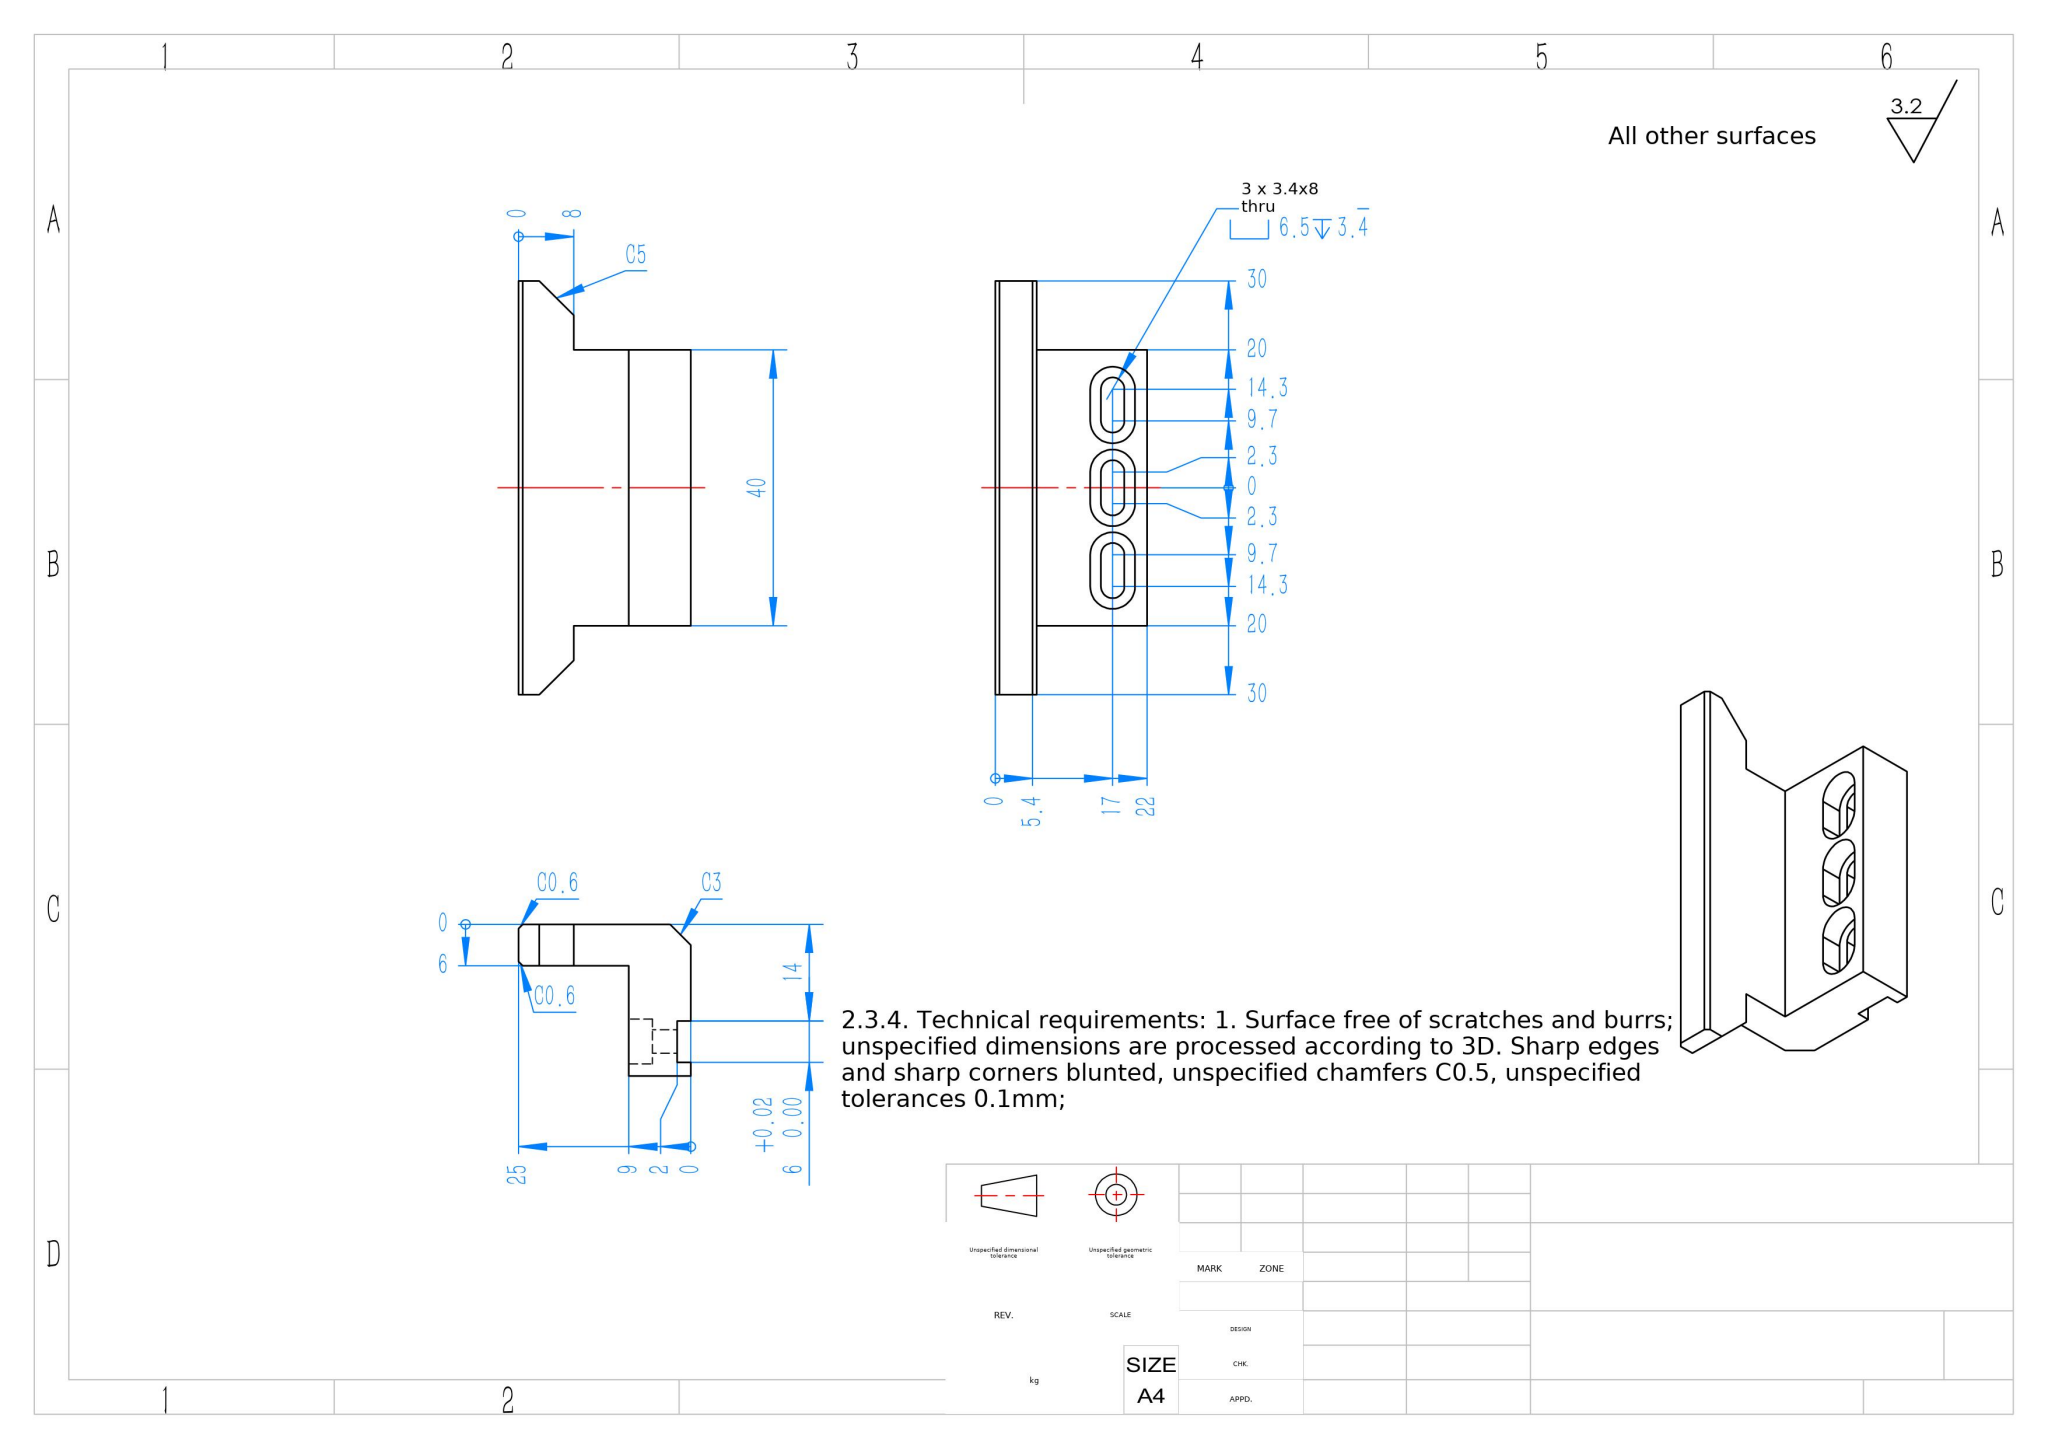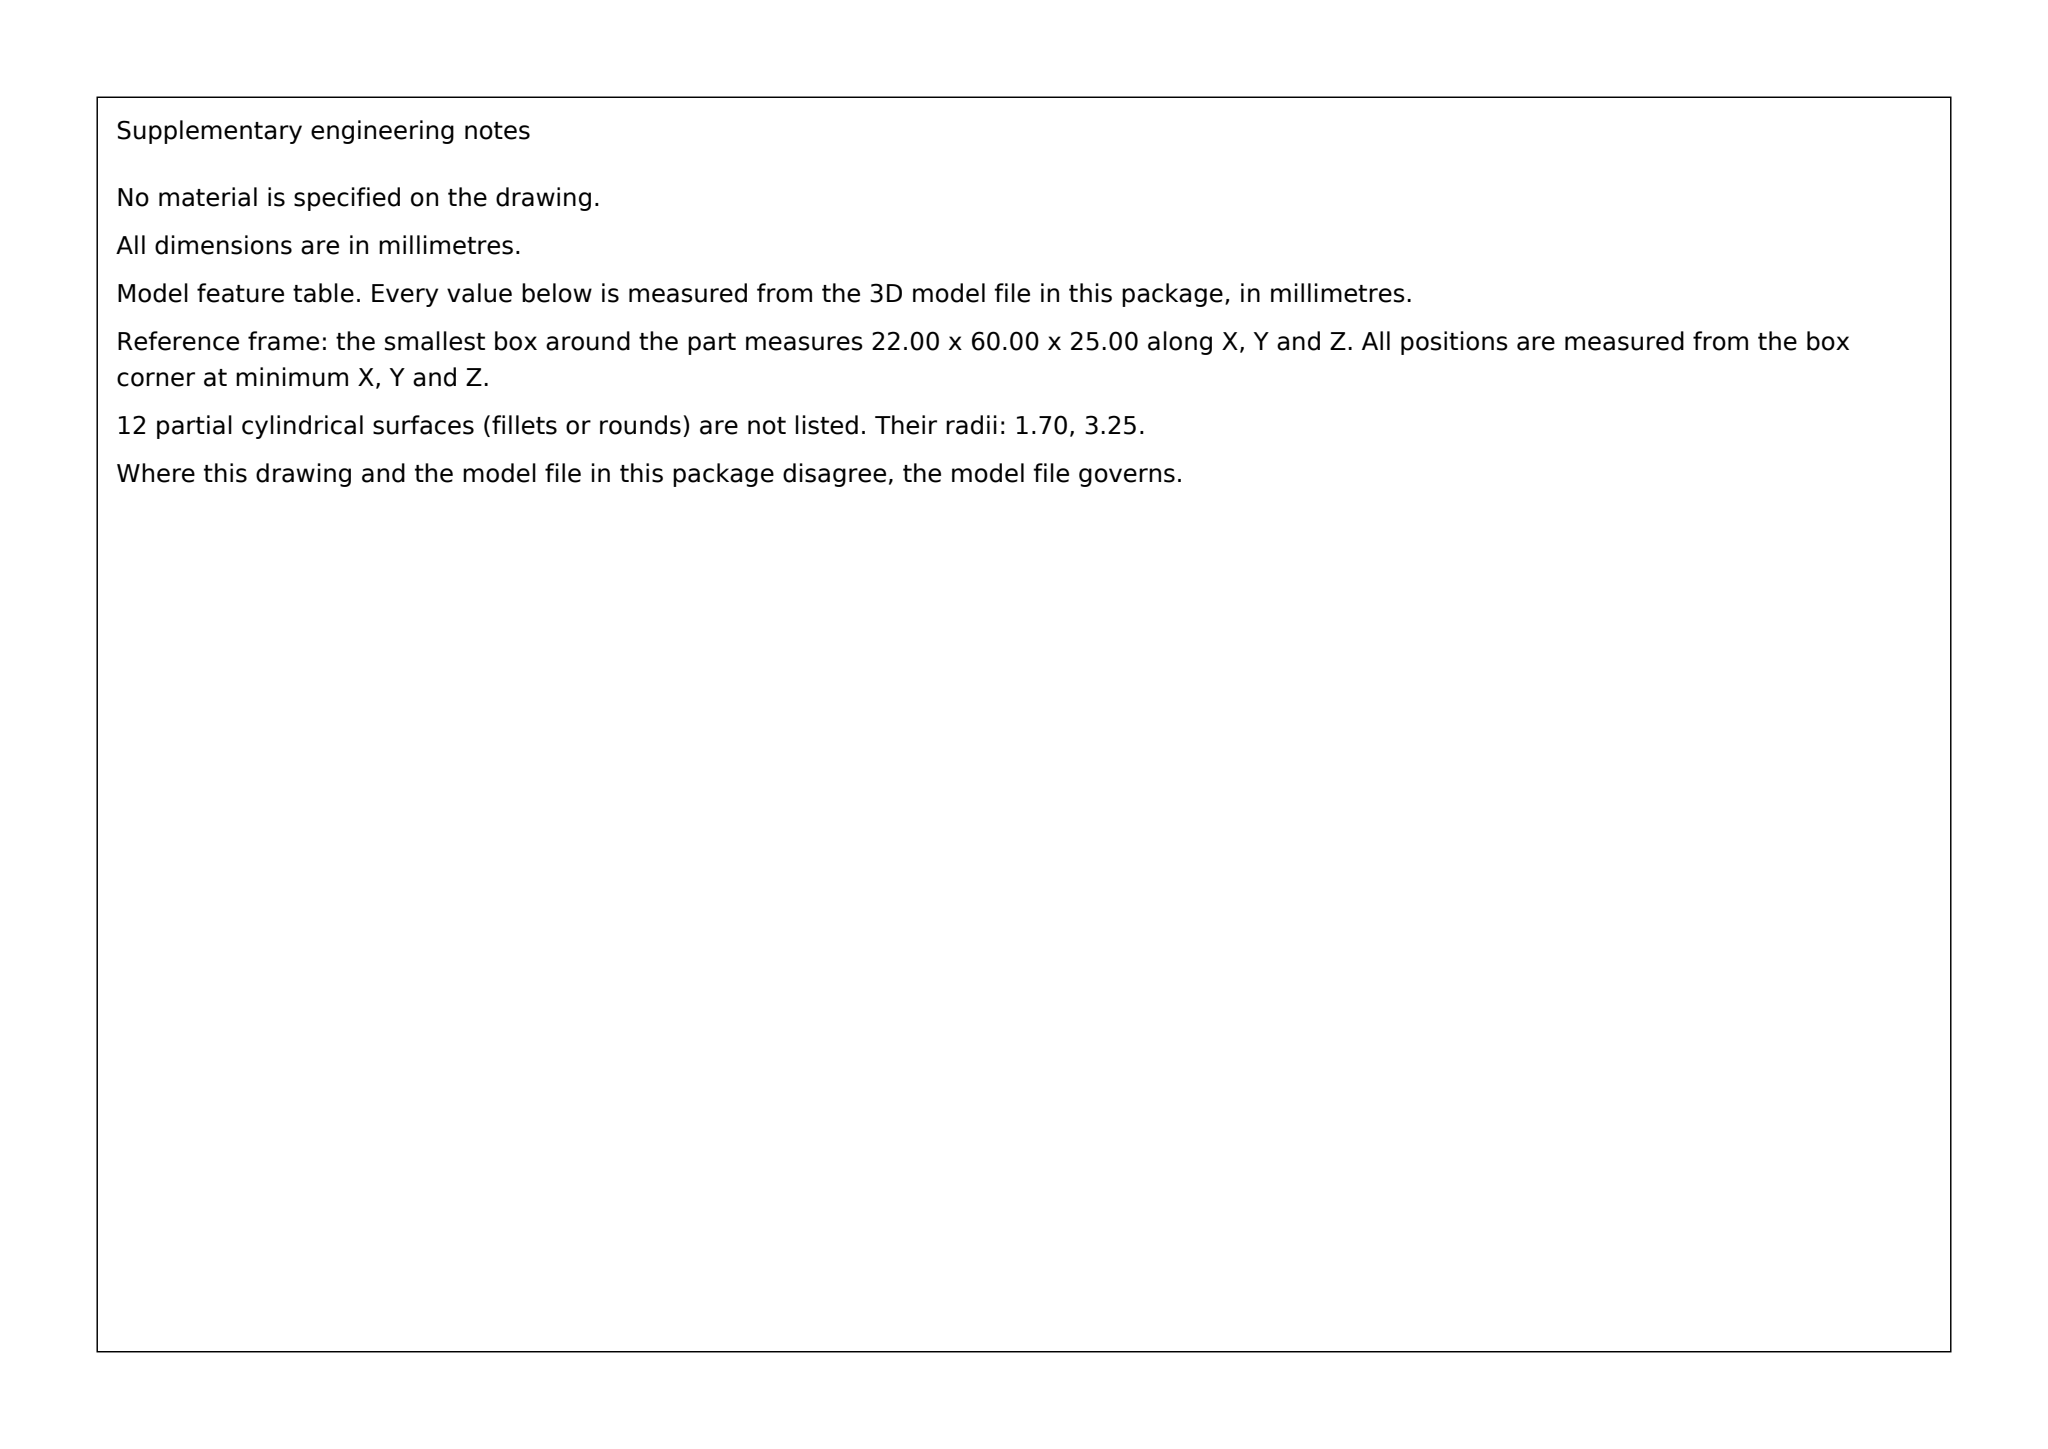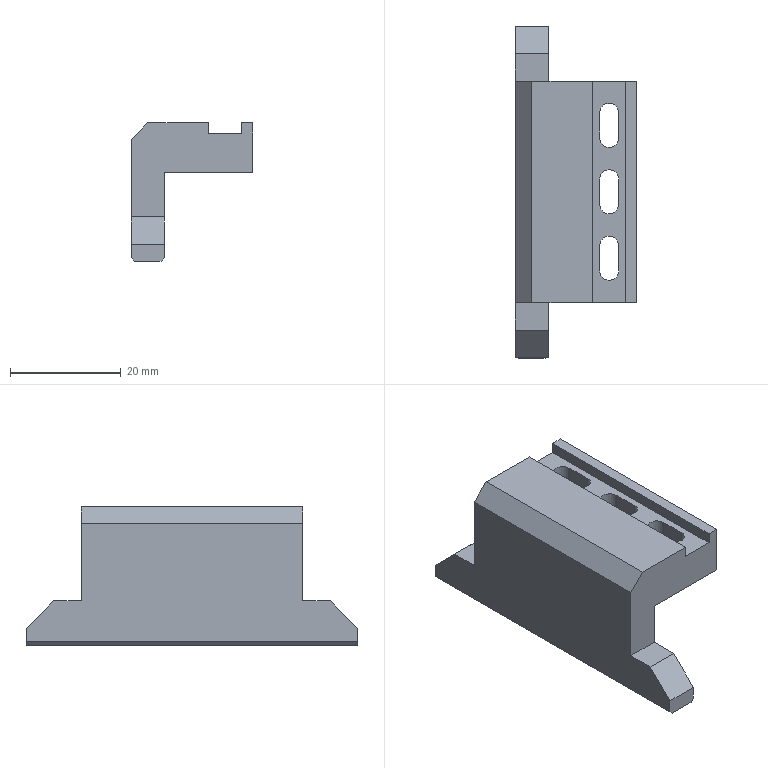Part | SolidWorks | mm | 1 solid | 48 faces | box 22 x 60 x 25 mm | volume 10978 mm3 | plane 36 | cylinder 12 | commonest cylinder face diameters 3.4 x6 6.5 x6